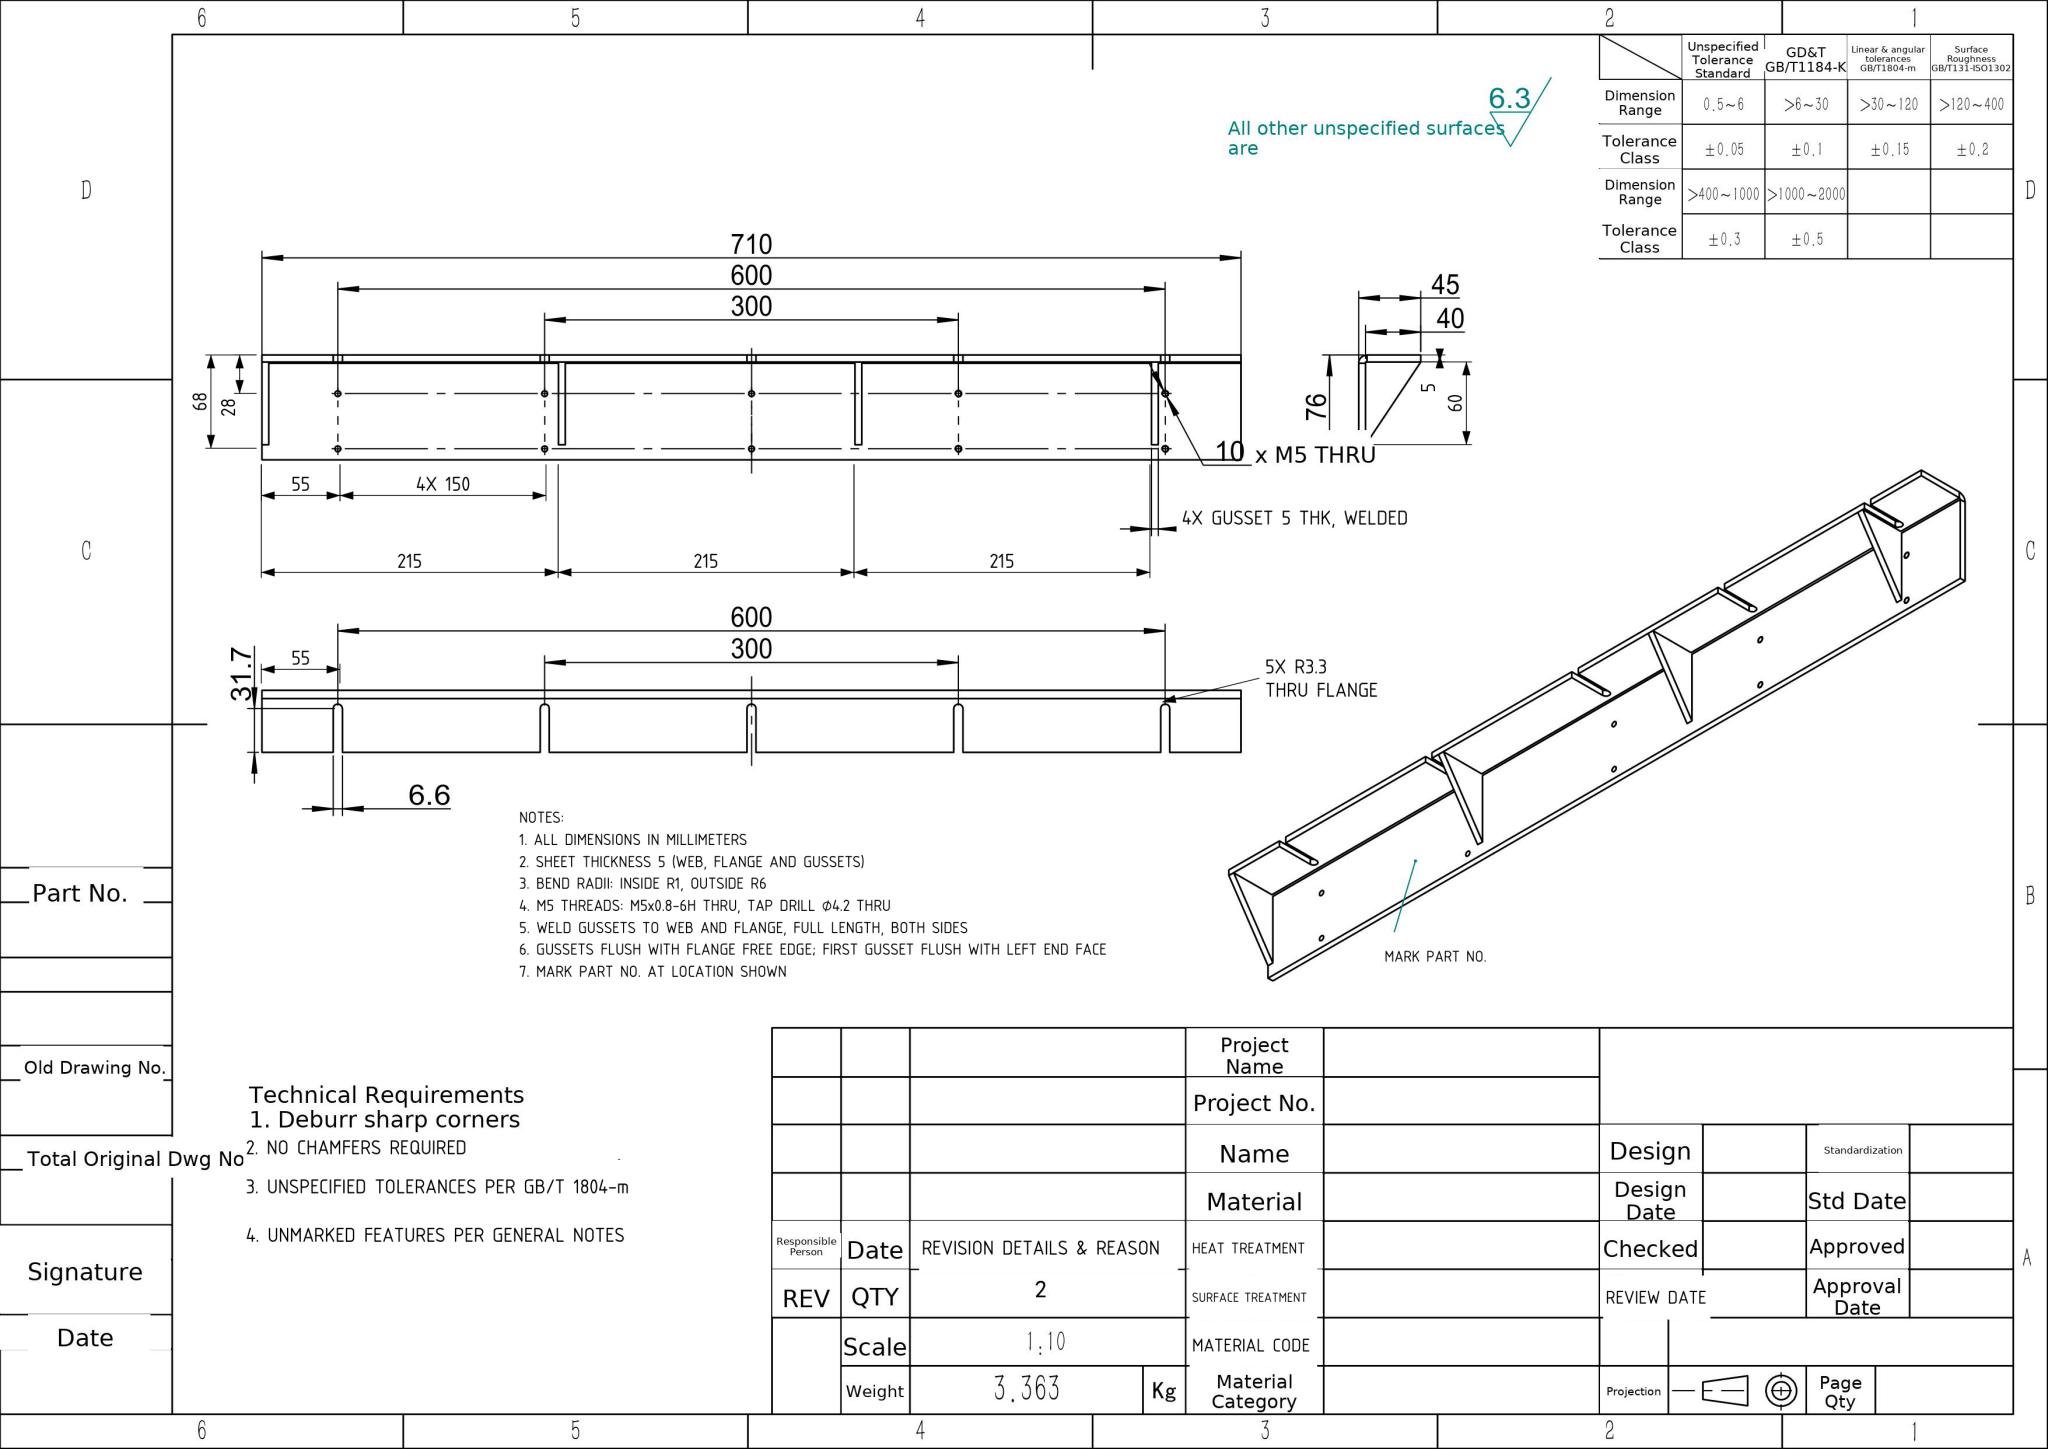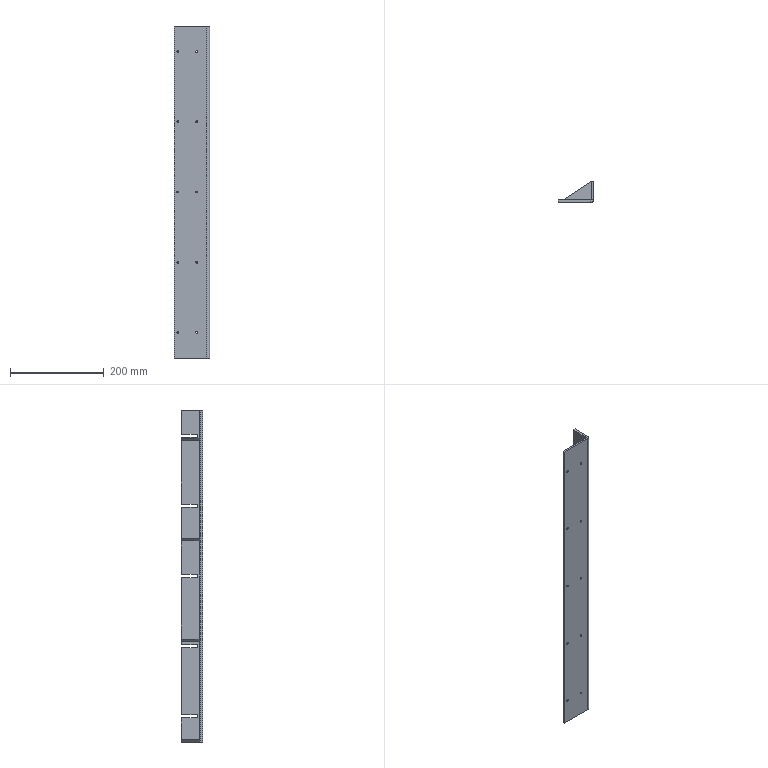Part | NX | mm | 1 solid | 69 faces | box 76 x 45 x 710 mm | volume 424112 mm3 | plane 39 | cylinder 30 | commonest cylinder face diameters 4.2 x20 6.6 x5 2 x4 12 x1